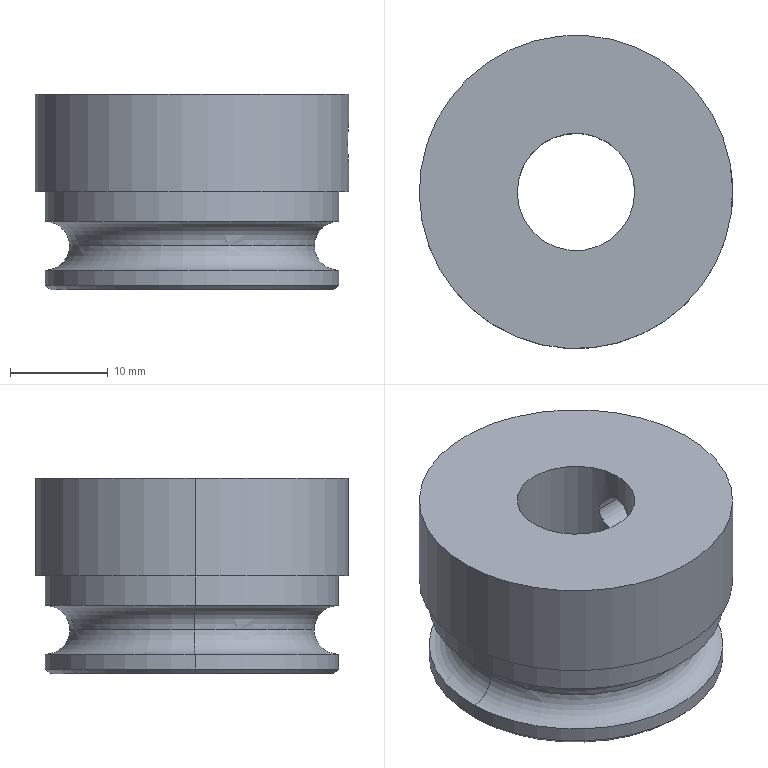Component | SolidWorks | TAR-02-032SmallPulley-1 | 1 solid | 19 faces | box 32 x 32 x 20 mm | volume 11838 mm3 | cylinder 10 | torus 4 | plane 3 | cone 2 | commonest cylinder face diameters 30 x4 4.2 x2 12 x2 32 x2
build123d program:
from build123d import *

# Parameters (mm, degrees)
CHAMFER1_SIZE         = 0.5
SKETCH2_R             = 16
BOSS_EXTRUDE1_DEPTH   = 10
SKETCH3_R             = 6
CUT_EXTRUDE1_DEPTH    = 99
M5_TAPPED_HOLE1_D     = 4.2
M5_TAPPED_HOLE1_DEPTH = 12.4
M5_TAPPED_HOLE1_TIP   = 1.262


with BuildPart() as part:
    # Sketch1 → Revolve1 (revolve)
    with BuildSketch(Plane.XY, mode=Mode.PRIVATE) as revolve1_sk:
        with BuildLine():
            Line((-21.881, 5.308), (-21.881, -9.692))
            Line((-21.881, -9.692), (-11.881, -9.692))
            Line((-11.881, -9.692), (-11.881, 5.308))
            Line((-11.881, 5.308), (-13.881, 5.308))
            ThreePointArc((-13.881, 5.308), (-16.381, 2.808), (-18.881, 5.308))
            Line((-18.881, 5.308), (-21.881, 5.308))
        make_face()
    revolve(revolve1_sk.sketch.rotate(Axis((-21.881, -9.692, 0), (1, 0, 0)), 90), axis=Axis((-21.881, -9.692, 0), (1, 0, 0)))

    # Chamfer1
    chamfer1_edges = [part.edges().sort_by_distance(p)[0] for p in [
        (-11.881, -9.692, -15),
    ]]
    chamfer(chamfer1_edges, length=CHAMFER1_SIZE)

    # Sketch2 → Boss-Extrude1 (add)
    with BuildSketch(Plane.ZY.offset(21.881)):
        with Locations((0, -9.692)):
            Circle(SKETCH2_R)
    extrude(amount=BOSS_EXTRUDE1_DEPTH)

    # Sketch3 → Cut-Extrude1 (cut)
    with BuildSketch(Plane(origin=(-11.881, 0, 0), x_dir=(0, 0, -1), z_dir=(1, 0, 0))):
        with Locations((0, -9.692)):
            Circle(SKETCH3_R)
    extrude(amount=-CUT_EXTRUDE1_DEPTH, mode=Mode.SUBTRACT)

    # M5 Tapped Hole1
    with Locations(Plane(origin=(-26.881, -9.692, 16), x_dir=(0, 1, 0), z_dir=(0, 0, 1))):
        with Locations((0, 0)):
            Hole(M5_TAPPED_HOLE1_D / 2, depth=M5_TAPPED_HOLE1_DEPTH)
            with Locations((0, 0, -(M5_TAPPED_HOLE1_DEPTH + M5_TAPPED_HOLE1_TIP / 2))):  # 118° drill point
                Cone(0, M5_TAPPED_HOLE1_D / 2, M5_TAPPED_HOLE1_TIP, mode=Mode.SUBTRACT)


solid = part.part

# Placed as in the assembly
solid = solid.moved(Location((-115.595, 18.978, -50.504), (-89.996, 88.793, 89.996)))
STEP:
#1=CARTESIAN_POINT('',(-3.953,0.3781,-1.245));
#2=VERTEX_POINT('',#1);
#3=CARTESIAN_POINT('',(-4.051,0.376,-1.343));
#4=VERTEX_POINT('',#3);
#5=CARTESIAN_POINT('',(-3.953,0.3781,-1.343));
#6=DIRECTION('',(0.02107,-0.9998,0.));
#7=DIRECTION('',(0.9998,0.02107,0.));
#8=AXIS2_PLACEMENT_3D('',#5,#6,#7);
#9=CIRCLE('',#8,0.09843);
#10=EDGE_CURVE('',#2,#4,#9,.T.);
#11=ORIENTED_EDGE('',*,*,#10,.T.);
#12=CARTESIAN_POINT('',(-5.035,0.3553,-1.343));
#13=VERTEX_POINT('',#12);
#14=CARTESIAN_POINT('',(-4.543,0.3657,-1.343));
#15=DIRECTION('',(0.,0.,1.));
#16=DIRECTION('',(1.,0.,0.));
#17=AXIS2_PLACEMENT_3D('',#14,#15,#16);
#18=CIRCLE('',#17,0.4921);
#19=EDGE_CURVE('',#4,#13,#18,.T.);
#20=ORIENTED_EDGE('',*,*,#19,.T.);
#21=CARTESIAN_POINT('',(-5.133,0.3532,-1.245));
#22=VERTEX_POINT('',#21);
#23=CARTESIAN_POINT('',(-5.133,0.3532,-1.343));
#24=DIRECTION('',(-0.02107,0.9998,0.));
#25=DIRECTION('',(-0.9998,-0.02107,0.));
#26=AXIS2_PLACEMENT_3D('',#23,#24,#25);
#27=CIRCLE('',#26,0.09843);
#28=EDGE_CURVE('',#22,#13,#27,.T.);
#29=ORIENTED_EDGE('',*,*,#28,.F.);
#30=CARTESIAN_POINT('',(-4.543,0.3657,-1.245));
#31=DIRECTION('',(0.,0.,1.));
#32=DIRECTION('',(0.9998,0.02107,0.));
#33=AXIS2_PLACEMENT_3D('',#30,#31,#32);
#34=CIRCLE('',#33,0.5906);
#35=EDGE_CURVE('',#2,#22,#34,.T.);
#36=ORIENTED_EDGE('',*,*,#35,.F.);
#37=EDGE_LOOP('',(#11,#20,#29,#36));
#38=FACE_OUTER_BOUND('',#37,.T.);
#39=CARTESIAN_POINT('',(-4.543,0.3657,-1.343));
#40=DIRECTION('',(0.,0.,1.));
#41=DIRECTION('',(0.9998,0.02107,0.));
#42=AXIS2_PLACEMENT_3D('',#39,#40,#41);
#43=TOROIDAL_SURFACE('',#42,0.5906,0.09843);
#44=ADVANCED_FACE('',(#38),#43,.F.);
#45=ORIENTED_EDGE('',*,*,#28,.T.);
#46=CARTESIAN_POINT('',(-4.543,0.3657,-1.343));
#47=DIRECTION('',(0.,0.,1.));
#48=DIRECTION('',(1.,0.,0.));
#49=AXIS2_PLACEMENT_3D('',#46,#47,#48);
#50=CIRCLE('',#49,0.4921);
#51=EDGE_CURVE('',#13,#4,#50,.T.);
#52=ORIENTED_EDGE('',*,*,#51,.T.);
#53=ORIENTED_EDGE('',*,*,#10,.F.);
#54=CARTESIAN_POINT('',(-4.543,0.3657,-1.245));
#55=DIRECTION('',(0.,0.,1.));
#56=DIRECTION('',(0.9998,0.02107,0.));
#57=AXIS2_PLACEMENT_3D('',#54,#55,#56);
#58=CIRCLE('',#57,0.5906);
#59=EDGE_CURVE('',#22,#2,#58,.T.);
#60=ORIENTED_EDGE('',*,*,#59,.F.);
#61=EDGE_LOOP('',(#45,#52,#53,#60));
#62=FACE_OUTER_BOUND('',#61,.T.);
#63=CARTESIAN_POINT('',(-4.543,0.3657,-1.343));
#64=DIRECTION('',(0.,0.,1.));
#65=DIRECTION('',(0.9998,0.02107,0.));
#66=AXIS2_PLACEMENT_3D('',#63,#64,#65);
#67=TOROIDAL_SURFACE('',#66,0.5906,0.09843);
#68=ADVANCED_FACE('',(#62),#67,.F.);
#69=CARTESIAN_POINT('',(-4.323,0.453,-0.93));
#70=VERTEX_POINT('',#69);
#71=CARTESIAN_POINT('',(-4.307,0.3706,-0.8474));
#72=VERTEX_POINT('',#71);
#73=CARTESIAN_POINT('',(-4.323,0.453,-0.93));
#74=CARTESIAN_POINT('',(-4.323,0.453,-0.9246));
#75=CARTESIAN_POINT('',(-4.323,0.4524,-0.9192));
#76=CARTESIAN_POINT('',(-4.322,0.4503,-0.9084));
#77=CARTESIAN_POINT('',(-4.322,0.4487,-0.9033));
#78=CARTESIAN_POINT('',(-4.32,0.4446,-0.8933));
#79=CARTESIAN_POINT('',(-4.319,0.442,-0.8885));
#80=CARTESIAN_POINT('',(-4.317,0.4361,-0.8795));
#81=CARTESIAN_POINT('',(-4.316,0.4327,-0.8754));
#82=CARTESIAN_POINT('',(-4.313,0.4213,-0.864));
#83=CARTESIAN_POINT('',(-4.311,0.4124,-0.8579));
#84=CARTESIAN_POINT('',(-4.309,0.3974,-0.8516));
#85=CARTESIAN_POINT('',(-4.308,0.3922,-0.8501));
#86=CARTESIAN_POINT('',(-4.307,0.3816,-0.8479));
#87=CARTESIAN_POINT('',(-4.307,0.3761,-0.8474));
#88=CARTESIAN_POINT('',(-4.307,0.3706,-0.8474));
#89=B_SPLINE_CURVE_WITH_KNOTS('',3,(#73,#74,#75,#76,#77,#78,#79,#80,#81,#82,#83,#84,#85,#86,#87,#88),.UNSPECIFIED.,.F.,.F.,(4,2,2,2,2,2,2,4),(0.006618,0.007032,0.007445,0.007859,0.008272,0.009099,0.009512,0.009926),.UNSPECIFIED.);
#90=EDGE_CURVE('',#70,#72,#89,.T.);
#91=ORIENTED_EDGE('',*,*,#90,.F.);
#92=CARTESIAN_POINT('',(-3.92,0.4615,-0.93));
#93=VERTEX_POINT('',#92);
#94=CARTESIAN_POINT('',(-3.915,0.4616,-0.93));
#95=DIRECTION('',(0.9998,0.02107,0.));
#96=VECTOR('',#95,39.37);
#97=LINE('',#94,#96);
#98=EDGE_CURVE('',#70,#93,#97,.T.);
#99=ORIENTED_EDGE('',*,*,#98,.T.);
#100=CARTESIAN_POINT('',(-3.913,0.3789,-0.8474));
#101=VERTEX_POINT('',#100);
#102=CARTESIAN_POINT('',(-3.913,0.3789,-0.8474));
#103=CARTESIAN_POINT('',(-3.913,0.3843,-0.8474));
#104=CARTESIAN_POINT('',(-3.913,0.3898,-0.8479));
#105=CARTESIAN_POINT('',(-3.914,0.4004,-0.85));
#106=CARTESIAN_POINT('',(-3.914,0.4055,-0.8516));
#107=CARTESIAN_POINT('',(-3.915,0.4156,-0.8557));
#108=CARTESIAN_POINT('',(-3.915,0.4204,-0.8583));
#109=CARTESIAN_POINT('',(-3.916,0.4293,-0.8643));
#110=CARTESIAN_POINT('',(-3.917,0.4335,-0.8677));
#111=CARTESIAN_POINT('',(-3.918,0.4412,-0.8754));
#112=CARTESIAN_POINT('',(-3.918,0.4446,-0.8796));
#113=CARTESIAN_POINT('',(-3.919,0.4505,-0.8886));
#114=CARTESIAN_POINT('',(-3.919,0.4531,-0.8934));
#115=CARTESIAN_POINT('',(-3.92,0.4573,-0.9034));
#116=CARTESIAN_POINT('',(-3.92,0.4588,-0.9086));
#117=CARTESIAN_POINT('',(-3.92,0.4609,-0.9192));
#118=CARTESIAN_POINT('',(-3.92,0.4615,-0.9247));
#119=CARTESIAN_POINT('',(-3.92,0.4615,-0.93));
#120=B_SPLINE_CURVE_WITH_KNOTS('',3,(#102,#103,#104,#105,#106,#107,#108,#109,#110,#111,#112,#113,#114,#115,#116,#117,#118,#119),.UNSPECIFIED.,.F.,.F.,(4,2,2,2,2,2,2,2,4),(0.003287,0.003698,0.004108,0.004519,0.00493,0.005341,0.005751,0.006162,0.006573),.UNSPECIFIED.);
#121=EDGE_CURVE('',#101,#93,#120,.T.);
#122=ORIENTED_EDGE('',*,*,#121,.F.);
#123=CARTESIAN_POINT('',(-3.917,0.2962,-0.93));
#124=VERTEX_POINT('',#123);
#125=CARTESIAN_POINT('',(-3.917,0.2962,-0.93));
#126=CARTESIAN_POINT('',(-3.917,0.2962,-0.9246));
#127=CARTESIAN_POINT('',(-3.917,0.2967,-0.9192));
#128=CARTESIAN_POINT('',(-3.917,0.2988,-0.9086));
#129=CARTESIAN_POINT('',(-3.916,0.3004,-0.9034));
#130=CARTESIAN_POINT('',(-3.916,0.3046,-0.8934));
#131=CARTESIAN_POINT('',(-3.916,0.3071,-0.8886));
#132=CARTESIAN_POINT('',(-3.915,0.3131,-0.8796));
#133=CARTESIAN_POINT('',(-3.915,0.3166,-0.8754));
#134=CARTESIAN_POINT('',(-3.914,0.3281,-0.8639));
#135=CARTESIAN_POINT('',(-3.914,0.3373,-0.8578));
#136=CARTESIAN_POINT('',(-3.913,0.3572,-0.8495));
#137=CARTESIAN_POINT('',(-3.913,0.3681,-0.8474));
#138=CARTESIAN_POINT('',(-3.913,0.3789,-0.8474));
#139=B_SPLINE_CURVE_WITH_KNOTS('',3,(#125,#126,#127,#128,#129,#130,#131,#132,#133,#134,#135,#136,#137,#138),.UNSPECIFIED.,.F.,.F.,(4,2,2,2,2,2,4),(0.,0.0004109,0.0008218,0.001233,0.001644,0.002465,0.003287),.UNSPECIFIED.);
#140=EDGE_CURVE('',#124,#101,#139,.T.);
#141=ORIENTED_EDGE('',*,*,#140,.F.);
#142=CARTESIAN_POINT('',(-4.32,0.2877,-0.93));
#143=VERTEX_POINT('',#142);
#144=CARTESIAN_POINT('',(-3.911,0.2963,-0.93));
#145=DIRECTION('',(0.9998,0.02107,0.));
#146=VECTOR('',#145,39.37);
#147=LINE('',#144,#146);
#148=EDGE_CURVE('',#143,#124,#147,.T.);
#149=ORIENTED_EDGE('',*,*,#148,.F.);
#150=CARTESIAN_POINT('',(-4.307,0.3706,-0.8474));
#151=CARTESIAN_POINT('',(-4.307,0.3652,-0.8474));
#152=CARTESIAN_POINT('',(-4.307,0.3598,-0.8479));
#153=CARTESIAN_POINT('',(-4.307,0.3491,-0.85));
#154=CARTESIAN_POINT('',(-4.308,0.3438,-0.8517));
#155=CARTESIAN_POINT('',(-4.309,0.3288,-0.8579));
#156=CARTESIAN_POINT('',(-4.311,0.3196,-0.864));
#157=CARTESIAN_POINT('',(-4.314,0.3082,-0.8754));
#158=CARTESIAN_POINT('',(-4.315,0.3047,-0.8796));
#159=CARTESIAN_POINT('',(-4.316,0.2987,-0.8885));
#160=CARTESIAN_POINT('',(-4.317,0.2962,-0.8933));
#161=CARTESIAN_POINT('',(-4.319,0.292,-0.9033));
#162=CARTESIAN_POINT('',(-4.319,0.2903,-0.9085));
#163=CARTESIAN_POINT('',(-4.32,0.2882,-0.9191));
#164=CARTESIAN_POINT('',(-4.32,0.2877,-0.9245));
#165=CARTESIAN_POINT('',(-4.32,0.2877,-0.93));
#166=B_SPLINE_CURVE_WITH_KNOTS('',3,(#150,#151,#152,#153,#154,#155,#156,#157,#158,#159,#160,#161,#162,#163,#164,#165),.UNSPECIFIED.,.F.,.F.,(4,2,2,2,2,2,2,4),(0.009926,0.01034,0.01075,0.01158,0.01199,0.01241,0.01282,0.01323),.UNSPECIFIED.);
#167=EDGE_CURVE('',#72,#143,#166,.T.);
#168=ORIENTED_EDGE('',*,*,#167,.F.);
#169=EDGE_LOOP('',(#91,#99,#122,#141,#149,#168));
#170=FACE_OUTER_BOUND('',#169,.T.);
#171=CARTESIAN_POINT('',(-3.913,0.3789,-0.93));
#172=DIRECTION('',(0.9998,0.02107,0.));
#173=DIRECTION('',(0.02107,-0.9998,0.));
#174=AXIS2_PLACEMENT_3D('',#171,#172,#173);
#175=CYLINDRICAL_SURFACE('',#174,0.08268);
#176=ADVANCED_FACE('',(#170),#175,.F.);
#177=CARTESIAN_POINT('',(-4.779,0.3607,-0.7332));
#178=VERTEX_POINT('',#177);
#179=CARTESIAN_POINT('',(-4.307,0.3706,-0.7332));
#180=VERTEX_POINT('',#179);
#181=CARTESIAN_POINT('',(-4.543,0.3657,-0.7332));
#182=DIRECTION('',(0.,0.,1.));
#183=DIRECTION('',(0.9998,0.02107,0.));
#184=AXIS2_PLACEMENT_3D('',#181,#182,#183);
#185=CIRCLE('',#184,0.2362);
#186=EDGE_CURVE('',#178,#180,#185,.T.);
#187=ORIENTED_EDGE('',*,*,#186,.T.);
#188=CARTESIAN_POINT('',(-4.307,0.3706,2.377));
#189=DIRECTION('',(0.,0.,-1.));
#190=VECTOR('',#189,39.37);
#191=LINE('',#188,#190);
#192=EDGE_CURVE('',#180,#72,#191,.T.);
#193=ORIENTED_EDGE('',*,*,#192,.T.);
#194=ORIENTED_EDGE('',*,*,#167,.T.);
#195=CARTESIAN_POINT('',(-4.307,0.3706,-1.013));
#196=VERTEX_POINT('',#195);
#197=CARTESIAN_POINT('',(-4.32,0.2877,-0.93));
#198=CARTESIAN_POINT('',(-4.32,0.2877,-0.9356));
#199=CARTESIAN_POINT('',(-4.32,0.2882,-0.941));
#200=CARTESIAN_POINT('',(-4.319,0.2904,-0.9516));
#201=CARTESIAN_POINT('',(-4.319,0.292,-0.9569));
#202=CARTESIAN_POINT('',(-4.317,0.2962,-0.9669));
#203=CARTESIAN_POINT('',(-4.316,0.2987,-0.9716));
#204=CARTESIAN_POINT('',(-4.315,0.3048,-0.9806));
#205=CARTESIAN_POINT('',(-4.314,0.3082,-0.9848));
#206=CARTESIAN_POINT('',(-4.311,0.3197,-0.9961));
#207=CARTESIAN_POINT('',(-4.309,0.3289,-1.002));
#208=CARTESIAN_POINT('',(-4.308,0.3438,-1.008));
#209=CARTESIAN_POINT('',(-4.307,0.3491,-1.01));
#210=CARTESIAN_POINT('',(-4.307,0.3598,-1.012));
#211=CARTESIAN_POINT('',(-4.307,0.3652,-1.013));
#212=CARTESIAN_POINT('',(-4.307,0.3706,-1.013));
#213=B_SPLINE_CURVE_WITH_KNOTS('',3,(#197,#198,#199,#200,#201,#202,#203,#204,#205,#206,#207,#208,#209,#210,#211,#212),.UNSPECIFIED.,.F.,.F.,(4,2,2,2,2,2,2,4),(0.,0.0004138,0.0008275,0.001241,0.001655,0.002483,0.002896,0.00331),.UNSPECIFIED.);
#214=EDGE_CURVE('',#143,#196,#213,.T.);
#215=ORIENTED_EDGE('',*,*,#214,.T.);
#216=CARTESIAN_POINT('',(-4.307,0.3706,-1.521));
#217=VERTEX_POINT('',#216);
#218=CARTESIAN_POINT('',(-4.307,0.3706,2.377));
#219=DIRECTION('',(0.,0.,-1.));
#220=VECTOR('',#219,39.37);
#221=LINE('',#218,#220);
#222=EDGE_CURVE('',#196,#217,#221,.T.);
#223=ORIENTED_EDGE('',*,*,#222,.T.);
#224=CARTESIAN_POINT('',(-4.779,0.3607,-1.521));
#225=VERTEX_POINT('',#224);
#226=CARTESIAN_POINT('',(-4.543,0.3657,-1.521));
#227=DIRECTION('',(0.,0.,-1.));
#228=DIRECTION('',(-0.9998,-0.02107,0.));
#229=AXIS2_PLACEMENT_3D('',#226,#227,#228);
#230=CIRCLE('',#229,0.2362);
#231=EDGE_CURVE('',#217,#225,#230,.T.);
#232=ORIENTED_EDGE('',*,*,#231,.T.);
#233=CARTESIAN_POINT('',(-4.779,0.3607,2.377));
#234=DIRECTION('',(0.,0.,-1.));
#235=VECTOR('',#234,39.37);
#236=LINE('',#233,#235);
#237=EDGE_CURVE('',#178,#225,#236,.T.);
#238=ORIENTED_EDGE('',*,*,#237,.F.);
#239=EDGE_LOOP('',(#187,#193,#194,#215,#223,#232,#238));
#240=FACE_OUTER_BOUND('',#239,.T.);
#241=CARTESIAN_POINT('',(-4.543,0.3657,2.377));
#242=DIRECTION('',(0.,0.,-1.));
#243=DIRECTION('',(-0.9998,-0.02107,0.));
#244=AXIS2_PLACEMENT_3D('',#241,#242,#243);
#245=CYLINDRICAL_SURFACE('',#244,0.2362);
#246=ADVANCED_FACE('',(#240),#245,.F.);
#247=CARTESIAN_POINT('',(-3.913,0.3789,-0.7332));
#248=VERTEX_POINT('',#247);
#249=CARTESIAN_POINT('',(-5.173,0.3524,-0.7332));
#250=VERTEX_POINT('',#249);
#251=CARTESIAN_POINT('',(-4.543,0.3657,-0.7332));
#252=DIRECTION('',(0.,0.,1.));
#253=DIRECTION('',(0.9998,0.02107,0.));
#254=AXIS2_PLACEMENT_3D('',#251,#252,#253);
#255=CIRCLE('',#254,0.6299);
#256=EDGE_CURVE('',#248,#250,#255,.T.);
#257=ORIENTED_EDGE('',*,*,#256,.F.);
#258=CARTESIAN_POINT('',(-3.913,0.3789,-0.7332));
#259=DIRECTION('',(0.,0.,-1.));
#260=VECTOR('',#259,39.37);
#261=LINE('',#258,#260);
#262=EDGE_CURVE('',#248,#101,#261,.T.);
#263=ORIENTED_EDGE('',*,*,#262,.T.);
#264=ORIENTED_EDGE('',*,*,#121,.T.);
#265=CARTESIAN_POINT('',(-3.913,0.3789,-1.013));
#266=VERTEX_POINT('',#265);
#267=CARTESIAN_POINT('',(-3.92,0.4615,-0.93));
#268=CARTESIAN_POINT('',(-3.92,0.4615,-0.9408));
#269=CARTESIAN_POINT('',(-3.92,0.4593,-0.9517));
#270=CARTESIAN_POINT('',(-3.919,0.4511,-0.9716));
#271=CARTESIAN_POINT('',(-3.918,0.4449,-0.9809));
#272=CARTESIAN_POINT('',(-3.917,0.4335,-0.9923));
#273=CARTESIAN_POINT('',(-3.916,0.4293,-0.9958));
#274=CARTESIAN_POINT('',(-3.915,0.4203,-1.002));
#275=CARTESIAN_POINT('',(-3.915,0.4156,-1.004));
#276=CARTESIAN_POINT('',(-3.914,0.4056,-1.008));
#277=CARTESIAN_POINT('',(-3.914,0.4003,-1.01));
#278=CARTESIAN_POINT('',(-3.913,0.3898,-1.012));
#279=CARTESIAN_POINT('',(-3.913,0.3844,-1.013));
#280=CARTESIAN_POINT('',(-3.913,0.3789,-1.013));
#281=B_SPLINE_CURVE_WITH_KNOTS('',3,(#267,#268,#269,#270,#271,#272,#273,#274,#275,#276,#277,#278,#279,#280),.UNSPECIFIED.,.F.,.F.,(4,2,2,2,2,2,4),(0.006573,0.007394,0.008216,0.008627,0.009038,0.009449,0.00986),.UNSPECIFIED.);
#282=EDGE_CURVE('',#93,#266,#281,.T.);
#283=ORIENTED_EDGE('',*,*,#282,.T.);
#284=CARTESIAN_POINT('',(-3.913,0.3789,-1.127));
#285=VERTEX_POINT('',#284);
#286=CARTESIAN_POINT('',(-3.913,0.3789,-0.7332));
#287=DIRECTION('',(0.,0.,-1.));
#288=VECTOR('',#287,39.37);
#289=LINE('',#286,#288);
#290=EDGE_CURVE('',#266,#285,#289,.T.);
#291=ORIENTED_EDGE('',*,*,#290,.T.);
#292=CARTESIAN_POINT('',(-5.173,0.3524,-1.127));
#293=VERTEX_POINT('',#292);
#294=CARTESIAN_POINT('',(-4.543,0.3657,-1.127));
#295=DIRECTION('',(0.,0.,1.));
#296=DIRECTION('',(0.9998,0.02107,0.));
#297=AXIS2_PLACEMENT_3D('',#294,#295,#296);
#298=CIRCLE('',#297,0.6299);
#299=EDGE_CURVE('',#285,#293,#298,.T.);
#300=ORIENTED_EDGE('',*,*,#299,.T.);
#301=CARTESIAN_POINT('',(-5.173,0.3524,-0.7332));
#302=DIRECTION('',(0.,0.,-1.));
#303=VECTOR('',#302,39.37);
#304=LINE('',#301,#303);
#305=EDGE_CURVE('',#250,#293,#304,.T.);
#306=ORIENTED_EDGE('',*,*,#305,.F.);
#307=EDGE_LOOP('',(#257,#263,#264,#283,#291,#300,#306));
#308=FACE_OUTER_BOUND('',#307,.T.);
#309=CARTESIAN_POINT('',(-4.543,0.3657,-0.7332));
#310=DIRECTION('',(0.,0.,-1.));
#311=DIRECTION('',(-0.9998,-0.02107,0.));
#312=AXIS2_PLACEMENT_3D('',#309,#310,#311);
#313=CYLINDRICAL_SURFACE('',#312,0.6299);
#314=ADVANCED_FACE('',(#308),#313,.T.);
#315=CARTESIAN_POINT('',(-5.114,0.3536,-1.521));
#316=VERTEX_POINT('',#315);
#317=CARTESIAN_POINT('',(-3.972,0.3777,-1.521));
#318=VERTEX_POINT('',#317);
#319=CARTESIAN_POINT('',(-4.543,0.3657,-1.521));
#320=DIRECTION('',(0.,0.,-1.));
#321=DIRECTION('',(0.9998,0.02107,0.));
#322=AXIS2_PLACEMENT_3D('',#319,#320,#321);
#323=CIRCLE('',#322,0.5709);
#324=EDGE_CURVE('',#316,#318,#323,.T.);
#325=ORIENTED_EDGE('',*,*,#324,.F.);
#326=CARTESIAN_POINT('',(-5.133,0.3532,-1.501));
#327=VERTEX_POINT('',#326);
#328=CARTESIAN_POINT('',(-5.133,0.3532,-1.501));
#329=DIRECTION('',(-0.7069,-0.0149,0.7071));
#330=VECTOR('',#329,39.37);
#331=LINE('',#328,#330);
#332=EDGE_CURVE('',#316,#327,#331,.T.);
#333=ORIENTED_EDGE('',*,*,#332,.T.);
#334=CARTESIAN_POINT('',(-3.953,0.3781,-1.501));
#335=VERTEX_POINT('',#334);
#336=CARTESIAN_POINT('',(-4.543,0.3657,-1.501));
#337=DIRECTION('',(0.,0.,1.));
#338=DIRECTION('',(0.9998,0.02107,0.));
#339=AXIS2_PLACEMENT_3D('',#336,#337,#338);
#340=CIRCLE('',#339,0.5906);
#341=EDGE_CURVE('',#335,#327,#340,.T.);
#342=ORIENTED_EDGE('',*,*,#341,.F.);
#343=CARTESIAN_POINT('',(-3.953,0.3781,-1.501));
#344=DIRECTION('',(0.7069,0.0149,0.7071));
#345=VECTOR('',#344,39.37);
#346=LINE('',#343,#345);
#347=EDGE_CURVE('',#318,#335,#346,.T.);
#348=ORIENTED_EDGE('',*,*,#347,.F.);
#349=EDGE_LOOP('',(#325,#333,#342,#348));
#350=FACE_OUTER_BOUND('',#349,.T.);
#351=CARTESIAN_POINT('',(-4.543,0.3657,-1.501));
#352=DIRECTION('',(0.,0.,1.));
#353=DIRECTION('',(0.9998,0.02107,0.));
#354=AXIS2_PLACEMENT_3D('',#351,#352,#353);
#355=CONICAL_SURFACE('',#354,0.5906,0.7854);
#356=ADVANCED_FACE('',(#350),#355,.T.);
#357=ORIENTED_EDGE('',*,*,#51,.F.);
#358=CARTESIAN_POINT('',(-5.133,0.3532,-1.442));
#359=VERTEX_POINT('',#358);
#360=CARTESIAN_POINT('',(-5.133,0.3532,-1.343));
#361=DIRECTION('',(-0.02107,0.9998,0.));
#362=DIRECTION('',(-0.9998,-0.02107,0.));
#363=AXIS2_PLACEMENT_3D('',#360,#361,#362);
#364=CIRCLE('',#363,0.09843);
#365=EDGE_CURVE('',#13,#359,#364,.T.);
#366=ORIENTED_EDGE('',*,*,#365,.T.);
#367=CARTESIAN_POINT('',(-3.953,0.3781,-1.442));
#368=VERTEX_POINT('',#367);
#369=CARTESIAN_POINT('',(-4.543,0.3657,-1.442));
#370=DIRECTION('',(0.,0.,1.));
#371=DIRECTION('',(0.9998,0.02107,0.));
#372=AXIS2_PLACEMENT_3D('',#369,#370,#371);
#373=CIRCLE('',#372,0.5906);
#374=EDGE_CURVE('',#359,#368,#373,.T.);
#375=ORIENTED_EDGE('',*,*,#374,.T.);
#376=CARTESIAN_POINT('',(-3.953,0.3781,-1.343));
#377=DIRECTION('',(0.02107,-0.9998,0.));
#378=DIRECTION('',(0.9998,0.02107,0.));
#379=AXIS2_PLACEMENT_3D('',#376,#377,#378);
#380=CIRCLE('',#379,0.09843);
#381=EDGE_CURVE('',#4,#368,#380,.T.);
#382=ORIENTED_EDGE('',*,*,#381,.F.);
#383=EDGE_LOOP('',(#357,#366,#375,#382));
#384=FACE_OUTER_BOUND('',#383,.T.);
#385=CARTESIAN_POINT('',(-4.543,0.3657,-1.343));
#386=DIRECTION('',(0.,0.,1.));
#387=DIRECTION('',(0.9998,0.02107,0.));
#388=AXIS2_PLACEMENT_3D('',#385,#386,#387);
#389=TOROIDAL_SURFACE('',#388,0.5906,0.09843);
#390=ADVANCED_FACE('',(#384),#389,.F.);
#391=ORIENTED_EDGE('',*,*,#341,.T.);
#392=CARTESIAN_POINT('',(-5.133,0.3532,-1.127));
#393=DIRECTION('',(0.,0.,1.));
#394=VECTOR('',#393,39.37);
#395=LINE('',#392,#394);
#396=EDGE_CURVE('',#327,#359,#395,.T.);
#397=ORIENTED_EDGE('',*,*,#396,.T.);
#398=CARTESIAN_POINT('',(-4.543,0.3657,-1.442));
#399=DIRECTION('',(0.,0.,1.));
#400=DIRECTION('',(0.9998,0.02107,0.));
#401=AXIS2_PLACEMENT_3D('',#398,#399,#400);
#402=CIRCLE('',#401,0.5906);
#403=EDGE_CURVE('',#368,#359,#402,.T.);
#404=ORIENTED_EDGE('',*,*,#403,.F.);
#405=CARTESIAN_POINT('',(-3.953,0.3781,-1.127));
#406=DIRECTION('',(0.,0.,1.));
#407=VECTOR('',#406,39.37);
#408=LINE('',#405,#407);
#409=EDGE_CURVE('',#335,#368,#408,.T.);
#410=ORIENTED_EDGE('',*,*,#409,.F.);
#411=EDGE_LOOP('',(#391,#397,#404,#410));
#412=FACE_OUTER_BOUND('',#411,.T.);
#413=CARTESIAN_POINT('',(-4.543,0.3657,-1.127));
#414=DIRECTION('',(0.,0.,1.));
#415=DIRECTION('',(0.9998,0.02107,0.));
#416=AXIS2_PLACEMENT_3D('',#413,#414,#415);
#417=CYLINDRICAL_SURFACE('',#416,0.5906);
#418=ADVANCED_FACE('',(#412),#417,.T.);
#419=ORIENTED_EDGE('',*,*,#35,.T.);
#420=CARTESIAN_POINT('',(-5.133,0.3532,-1.127));
#421=VERTEX_POINT('',#420);
#422=CARTESIAN_POINT('',(-5.133,0.3532,-1.127));
#423=DIRECTION('',(0.,0.,1.));
#424=VECTOR('',#423,39.37);
#425=LINE('',#422,#424);
#426=EDGE_CURVE('',#22,#421,#425,.T.);
#427=ORIENTED_EDGE('',*,*,#426,.T.);
#428=CARTESIAN_POINT('',(-3.953,0.3781,-1.127));
#429=VERTEX_POINT('',#428);
#430=CARTESIAN_POINT('',(-4.543,0.3657,-1.127));
#431=DIRECTION('',(0.,0.,1.));
#432=DIRECTION('',(0.9998,0.02107,0.));
#433=AXIS2_PLACEMENT_3D('',#430,#431,#432);
#434=CIRCLE('',#433,0.5906);
#435=EDGE_CURVE('',#429,#421,#434,.T.);
#436=ORIENTED_EDGE('',*,*,#435,.F.);
#437=CARTESIAN_POINT('',(-3.953,0.3781,-1.127));
#438=DIRECTION('',(0.,0.,1.));
#439=VECTOR('',#438,39.37);
#440=LINE('',#437,#439);
#441=EDGE_CURVE('',#2,#429,#440,.T.);
#442=ORIENTED_EDGE('',*,*,#441,.F.);
#443=EDGE_LOOP('',(#419,#427,#436,#442));
#444=FACE_OUTER_BOUND('',#443,.T.);
#445=CARTESIAN_POINT('',(-4.543,0.3657,-1.127));
#446=DIRECTION('',(0.,0.,1.));
#447=DIRECTION('',(0.9998,0.02107,0.));
#448=AXIS2_PLACEMENT_3D('',#445,#446,#447);
#449=CYLINDRICAL_SURFACE('',#448,0.5906);
#450=ADVANCED_FACE('',(#444),#449,.T.);
#451=ORIENTED_EDGE('',*,*,#426,.F.);
#452=ORIENTED_EDGE('',*,*,#59,.T.);
#453=ORIENTED_EDGE('',*,*,#441,.T.);
#454=CARTESIAN_POINT('',(-4.543,0.3657,-1.127));
#455=DIRECTION('',(0.,0.,1.));
#456=DIRECTION('',(0.9998,0.02107,0.));
#457=AXIS2_PLACEMENT_3D('',#454,#455,#456);
#458=CIRCLE('',#457,0.5906);
#459=EDGE_CURVE('',#421,#429,#458,.T.);
#460=ORIENTED_EDGE('',*,*,#459,.F.);
#461=EDGE_LOOP('',(#451,#452,#453,#460));
#462=FACE_OUTER_BOUND('',#461,.T.);
#463=CARTESIAN_POINT('',(-4.543,0.3657,-1.127));
#464=DIRECTION('',(0.,0.,1.));
#465=DIRECTION('',(0.9998,0.02107,0.));
#466=AXIS2_PLACEMENT_3D('',#463,#464,#465);
#467=CYLINDRICAL_SURFACE('',#466,0.5906);
#468=ADVANCED_FACE('',(#462),#467,.T.);
#469=CARTESIAN_POINT('',(-4.543,0.3657,-1.521));
#470=DIRECTION('',(0.,0.,-1.));
#471=DIRECTION('',(-0.9998,-0.02107,0.));
#472=AXIS2_PLACEMENT_3D('',#469,#470,#471);
#473=CIRCLE('',#472,0.2362);
#474=EDGE_CURVE('',#225,#217,#473,.T.);
#475=ORIENTED_EDGE('',*,*,#474,.F.);
#476=ORIENTED_EDGE('',*,*,#231,.F.);
#477=EDGE_LOOP('',(#475,#476));
#478=FACE_BOUND('',#477,.T.);
#479=CARTESIAN_POINT('',(-4.543,0.3657,-1.521));
#480=DIRECTION('',(0.,0.,-1.));
#481=DIRECTION('',(0.9998,0.02107,0.));
#482=AXIS2_PLACEMENT_3D('',#479,#480,#481);
#483=CIRCLE('',#482,0.5709);
#484=EDGE_CURVE('',#318,#316,#483,.T.);
#485=ORIENTED_EDGE('',*,*,#484,.T.);
#486=ORIENTED_EDGE('',*,*,#324,.T.);
#487=EDGE_LOOP('',(#485,#486));
#488=FACE_OUTER_BOUND('',#487,.T.);
#489=CARTESIAN_POINT('',(-4.543,0.3657,-1.521));
#490=DIRECTION('',(0.,0.,1.));
#491=DIRECTION('',(0.9998,0.02107,0.));
#492=AXIS2_PLACEMENT_3D('',#489,#490,#491);
#493=PLANE('',#492);
#494=ADVANCED_FACE('',(#478,#488),#493,.F.);
#495=ORIENTED_EDGE('',*,*,#396,.F.);
#496=CARTESIAN_POINT('',(-4.543,0.3657,-1.501));
#497=DIRECTION('',(0.,0.,1.));
#498=DIRECTION('',(0.9998,0.02107,0.));
#499=AXIS2_PLACEMENT_3D('',#496,#497,#498);
#500=CIRCLE('',#499,0.5906);
#501=EDGE_CURVE('',#327,#335,#500,.T.);
#502=ORIENTED_EDGE('',*,*,#501,.T.);
#503=ORIENTED_EDGE('',*,*,#409,.T.);
#504=ORIENTED_EDGE('',*,*,#374,.F.);
#505=EDGE_LOOP('',(#495,#502,#503,#504));
#506=FACE_OUTER_BOUND('',#505,.T.);
#507=CARTESIAN_POINT('',(-4.543,0.3657,-1.127));
#508=DIRECTION('',(0.,0.,1.));
#509=DIRECTION('',(0.9998,0.02107,0.));
#510=AXIS2_PLACEMENT_3D('',#507,#508,#509);
#511=CYLINDRICAL_SURFACE('',#510,0.5906);
#512=ADVANCED_FACE('',(#506),#511,.T.);
#513=ORIENTED_EDGE('',*,*,#19,.F.);
#514=ORIENTED_EDGE('',*,*,#381,.T.);
#515=ORIENTED_EDGE('',*,*,#403,.T.);
#516=ORIENTED_EDGE('',*,*,#365,.F.);
#517=EDGE_LOOP('',(#513,#514,#515,#516));
#518=FACE_OUTER_BOUND('',#517,.T.);
#519=CARTESIAN_POINT('',(-4.543,0.3657,-1.343));
#520=DIRECTION('',(0.,0.,1.));
#521=DIRECTION('',(0.9998,0.02107,0.));
#522=AXIS2_PLACEMENT_3D('',#519,#520,#521);
#523=TOROIDAL_SURFACE('',#522,0.5906,0.09843);
#524=ADVANCED_FACE('',(#518),#523,.F.);
#525=ORIENTED_EDGE('',*,*,#332,.F.);
#526=ORIENTED_EDGE('',*,*,#484,.F.);
#527=ORIENTED_EDGE('',*,*,#347,.T.);
#528=ORIENTED_EDGE('',*,*,#501,.F.);
#529=EDGE_LOOP('',(#525,#526,#527,#528));
#530=FACE_OUTER_BOUND('',#529,.T.);
#531=CARTESIAN_POINT('',(-4.543,0.3657,-1.501));
#532=DIRECTION('',(0.,0.,1.));
#533=DIRECTION('',(0.9998,0.02107,0.));
#534=AXIS2_PLACEMENT_3D('',#531,#532,#533);
#535=CONICAL_SURFACE('',#534,0.5906,0.7854);
#536=ADVANCED_FACE('',(#530),#535,.T.);
#537=ORIENTED_EDGE('',*,*,#262,.F.);
#538=CARTESIAN_POINT('',(-4.543,0.3657,-0.7332));
#539=DIRECTION('',(0.,0.,1.));
#540=DIRECTION('',(0.9998,0.02107,0.));
#541=AXIS2_PLACEMENT_3D('',#538,#539,#540);
#542=CIRCLE('',#541,0.6299);
#543=EDGE_CURVE('',#250,#248,#542,.T.);
#544=ORIENTED_EDGE('',*,*,#543,.F.);
#545=ORIENTED_EDGE('',*,*,#305,.T.);
#546=CARTESIAN_POINT('',(-4.543,0.3657,-1.127));
#547=DIRECTION('',(0.,0.,1.));
#548=DIRECTION('',(0.9998,0.02107,0.));
#549=AXIS2_PLACEMENT_3D('',#546,#547,#548);
#550=CIRCLE('',#549,0.6299);
#551=EDGE_CURVE('',#293,#285,#550,.T.);
#552=ORIENTED_EDGE('',*,*,#551,.T.);
#553=ORIENTED_EDGE('',*,*,#290,.F.);
#554=CARTESIAN_POINT('',(-3.913,0.3789,-1.013));
#555=CARTESIAN_POINT('',(-3.913,0.3735,-1.013));
#556=CARTESIAN_POINT('',(-3.913,0.3681,-1.012));
#557=CARTESIAN_POINT('',(-3.913,0.3575,-1.01));
#558=CARTESIAN_POINT('',(-3.913,0.3523,-1.008));
#559=CARTESIAN_POINT('',(-3.913,0.3423,-1.004));
#560=CARTESIAN_POINT('',(-3.914,0.3375,-1.002));
#561=CARTESIAN_POINT('',(-3.914,0.3285,-0.9958));
#562=CARTESIAN_POINT('',(-3.914,0.3243,-0.9923));
#563=CARTESIAN_POINT('',(-3.915,0.3128,-0.9809));
#564=CARTESIAN_POINT('',(-3.916,0.3066,-0.9717));
#565=CARTESIAN_POINT('',(-3.917,0.2984,-0.9518));
#566=CARTESIAN_POINT('',(-3.917,0.2962,-0.941));
#567=CARTESIAN_POINT('',(-3.917,0.2962,-0.93));
#568=B_SPLINE_CURVE_WITH_KNOTS('',3,(#554,#555,#556,#557,#558,#559,#560,#561,#562,#563,#564,#565,#566,#567),.UNSPECIFIED.,.F.,.F.,(4,2,2,2,2,2,4),(0.00986,0.01027,0.01068,0.01109,0.0115,0.01232,0.01314),.UNSPECIFIED.);
#569=EDGE_CURVE('',#266,#124,#568,.T.);
#570=ORIENTED_EDGE('',*,*,#569,.T.);
#571=ORIENTED_EDGE('',*,*,#140,.T.);
#572=EDGE_LOOP('',(#537,#544,#545,#552,#553,#570,#571));
#573=FACE_OUTER_BOUND('',#572,.T.);
#574=CARTESIAN_POINT('',(-4.543,0.3657,-0.7332));
#575=DIRECTION('',(0.,0.,-1.));
#576=DIRECTION('',(-0.9998,-0.02107,0.));
#577=AXIS2_PLACEMENT_3D('',#574,#575,#576);
#578=CYLINDRICAL_SURFACE('',#577,0.6299);
#579=ADVANCED_FACE('',(#573),#578,.T.);
#580=ORIENTED_EDGE('',*,*,#186,.F.);
#581=CARTESIAN_POINT('',(-4.543,0.3657,-0.7332));
#582=DIRECTION('',(0.,0.,1.));
#583=DIRECTION('',(0.9998,0.02107,0.));
#584=AXIS2_PLACEMENT_3D('',#581,#582,#583);
#585=CIRCLE('',#584,0.2362);
#586=EDGE_CURVE('',#180,#178,#585,.T.);
#587=ORIENTED_EDGE('',*,*,#586,.F.);
#588=EDGE_LOOP('',(#580,#587));
#589=FACE_BOUND('',#588,.T.);
#590=ORIENTED_EDGE('',*,*,#543,.T.);
#591=ORIENTED_EDGE('',*,*,#256,.T.);
#592=EDGE_LOOP('',(#590,#591));
#593=FACE_OUTER_BOUND('',#592,.T.);
#594=CARTESIAN_POINT('',(-4.543,0.3657,-0.7332));
#595=DIRECTION('',(0.,0.,1.));
#596=DIRECTION('',(0.9998,0.02107,0.));
#597=AXIS2_PLACEMENT_3D('',#594,#595,#596);
#598=PLANE('',#597);
#599=ADVANCED_FACE('',(#589,#593),#598,.T.);
#600=ORIENTED_EDGE('',*,*,#435,.T.);
#601=ORIENTED_EDGE('',*,*,#459,.T.);
#602=EDGE_LOOP('',(#600,#601));
#603=FACE_BOUND('',#602,.T.);
#604=ORIENTED_EDGE('',*,*,#551,.F.);
#605=ORIENTED_EDGE('',*,*,#299,.F.);
#606=EDGE_LOOP('',(#604,#605));
#607=FACE_OUTER_BOUND('',#606,.T.);
#608=CARTESIAN_POINT('',(-4.543,0.3657,-1.127));
#609=DIRECTION('',(0.,0.,1.));
#610=DIRECTION('',(0.9998,0.02107,0.));
#611=AXIS2_PLACEMENT_3D('',#608,#609,#610);
#612=PLANE('',#611);
#613=ADVANCED_FACE('',(#603,#607),#612,.F.);
#614=ORIENTED_EDGE('',*,*,#192,.F.);
#615=ORIENTED_EDGE('',*,*,#586,.T.);
#616=ORIENTED_EDGE('',*,*,#237,.T.);
#617=ORIENTED_EDGE('',*,*,#474,.T.);
#618=ORIENTED_EDGE('',*,*,#222,.F.);
#619=CARTESIAN_POINT('',(-4.307,0.3706,-1.013));
#620=CARTESIAN_POINT('',(-4.307,0.3761,-1.013));
#621=CARTESIAN_POINT('',(-4.307,0.3816,-1.012));
#622=CARTESIAN_POINT('',(-4.308,0.3922,-1.01));
#623=CARTESIAN_POINT('',(-4.309,0.3974,-1.008));
#624=CARTESIAN_POINT('',(-4.31,0.4074,-1.004));
#625=CARTESIAN_POINT('',(-4.311,0.4122,-1.002));
#626=CARTESIAN_POINT('',(-4.313,0.421,-0.9957));
#627=CARTESIAN_POINT('',(-4.314,0.4252,-0.9923));
#628=CARTESIAN_POINT('',(-4.316,0.4328,-0.9847));
#629=CARTESIAN_POINT('',(-4.317,0.4361,-0.9805));
#630=CARTESIAN_POINT('',(-4.319,0.4421,-0.9716));
#631=CARTESIAN_POINT('',(-4.32,0.4446,-0.9668));
#632=CARTESIAN_POINT('',(-4.322,0.4487,-0.9568));
#633=CARTESIAN_POINT('',(-4.322,0.4503,-0.9517));
#634=CARTESIAN_POINT('',(-4.323,0.4524,-0.941));
#635=CARTESIAN_POINT('',(-4.323,0.453,-0.9355));
#636=CARTESIAN_POINT('',(-4.323,0.453,-0.93));
#637=B_SPLINE_CURVE_WITH_KNOTS('',3,(#619,#620,#621,#622,#623,#624,#625,#626,#627,#628,#629,#630,#631,#632,#633,#634,#635,#636),.UNSPECIFIED.,.F.,.F.,(4,2,2,2,2,2,2,2,4),(0.00331,0.003724,0.004137,0.004551,0.004964,0.005378,0.005791,0.006205,0.006618),.UNSPECIFIED.);
#638=EDGE_CURVE('',#196,#70,#637,.T.);
#639=ORIENTED_EDGE('',*,*,#638,.T.);
#640=ORIENTED_EDGE('',*,*,#90,.T.);
#641=EDGE_LOOP('',(#614,#615,#616,#617,#618,#639,#640));
#642=FACE_OUTER_BOUND('',#641,.T.);
#643=CARTESIAN_POINT('',(-4.543,0.3657,2.377));
#644=DIRECTION('',(0.,0.,-1.));
#645=DIRECTION('',(-0.9998,-0.02107,0.));
#646=AXIS2_PLACEMENT_3D('',#643,#644,#645);
#647=CYLINDRICAL_SURFACE('',#646,0.2362);
#648=ADVANCED_FACE('',(#642),#647,.F.);
#649=ORIENTED_EDGE('',*,*,#98,.F.);
#650=ORIENTED_EDGE('',*,*,#638,.F.);
#651=ORIENTED_EDGE('',*,*,#214,.F.);
#652=ORIENTED_EDGE('',*,*,#148,.T.);
#653=ORIENTED_EDGE('',*,*,#569,.F.);
#654=ORIENTED_EDGE('',*,*,#282,.F.);
#655=EDGE_LOOP('',(#649,#650,#651,#652,#653,#654));
#656=FACE_OUTER_BOUND('',#655,.T.);
#657=CARTESIAN_POINT('',(-3.913,0.3789,-0.93));
#658=DIRECTION('',(0.9998,0.02107,0.));
#659=DIRECTION('',(0.02107,-0.9998,0.));
#660=AXIS2_PLACEMENT_3D('',#657,#658,#659);
#661=CYLINDRICAL_SURFACE('',#660,0.08268);
#662=ADVANCED_FACE('',(#656),#661,.F.);
#663=CLOSED_SHELL('',(#44,#68,#176,#246,#314,#356,#390,#418,#450,#468,#494,#512,#524,#536,#579,#599,#613,#648,#662));
#664=MANIFOLD_SOLID_BREP('',#663);
#665=CARTESIAN_POINT('',(0.,0.,0.));
#666=DIRECTION('',(0.,0.,1.));
#667=DIRECTION('',(1.,0.,0.));
#668=AXIS2_PLACEMENT_3D('',#665,#666,#667);
#669=(LENGTH_UNIT()NAMED_UNIT(*)SI_UNIT($,.METRE.));
#670=LENGTH_MEASURE_WITH_UNIT(LENGTH_MEASURE(0.0254),#669);
#671=DIMENSIONAL_EXPONENTS(1.,0.,0.,0.,0.,0.,0.);
#672=(CONVERSION_BASED_UNIT('',#670)LENGTH_UNIT()NAMED_UNIT(#671));
#673=UNCERTAINTY_MEASURE_WITH_UNIT(LENGTH_MEASURE(0.00001),#672,'','');
#674=(NAMED_UNIT(*)PLANE_ANGLE_UNIT()SI_UNIT($,.RADIAN.));
#675=(NAMED_UNIT(*)SI_UNIT($,.STERADIAN.)SOLID_ANGLE_UNIT());
#676=(GEOMETRIC_REPRESENTATION_CONTEXT(3)GLOBAL_UNCERTAINTY_ASSIGNED_CONTEXT((#673))GLOBAL_UNIT_ASSIGNED_CONTEXT((#672,#674,#675))REPRESENTATION_CONTEXT('',''));
#677=ADVANCED_BREP_SHAPE_REPRESENTATION('',(#664,#668),#676);
#678=COLOUR_RGB('',0.7922,0.8196,0.9333);
#679=FILL_AREA_STYLE_COLOUR('',#678);
#680=FILL_AREA_STYLE('',(#679));
#681=SURFACE_STYLE_FILL_AREA(#680);
#682=SURFACE_SIDE_STYLE('',(#681));
#683=SURFACE_STYLE_USAGE(.BOTH.,#682);
#684=PRESENTATION_STYLE_ASSIGNMENT((#683));
#685=STYLED_ITEM('',(#684),#664);
#686=(LENGTH_UNIT()NAMED_UNIT(*)SI_UNIT($,.METRE.));
#687=LENGTH_MEASURE_WITH_UNIT(LENGTH_MEASURE(0.0254),#686);
#688=DIMENSIONAL_EXPONENTS(1.,0.,0.,0.,0.,0.,0.);
#689=(CONVERSION_BASED_UNIT('',#687)LENGTH_UNIT()NAMED_UNIT(#688));
#690=UNCERTAINTY_MEASURE_WITH_UNIT(LENGTH_MEASURE(0.00001),#689,'','');
#691=(NAMED_UNIT(*)PLANE_ANGLE_UNIT()SI_UNIT($,.RADIAN.));
#692=(NAMED_UNIT(*)SI_UNIT($,.STERADIAN.)SOLID_ANGLE_UNIT());
#693=(GEOMETRIC_REPRESENTATION_CONTEXT(3)GLOBAL_UNCERTAINTY_ASSIGNED_CONTEXT((#690))GLOBAL_UNIT_ASSIGNED_CONTEXT((#689,#691,#692))REPRESENTATION_CONTEXT('',''));
#694=MECHANICAL_DESIGN_GEOMETRIC_PRESENTATION_REPRESENTATION('',(#685),#693);
#695=PRESENTATION_LAYER_ASSIGNMENT('','',(#685));